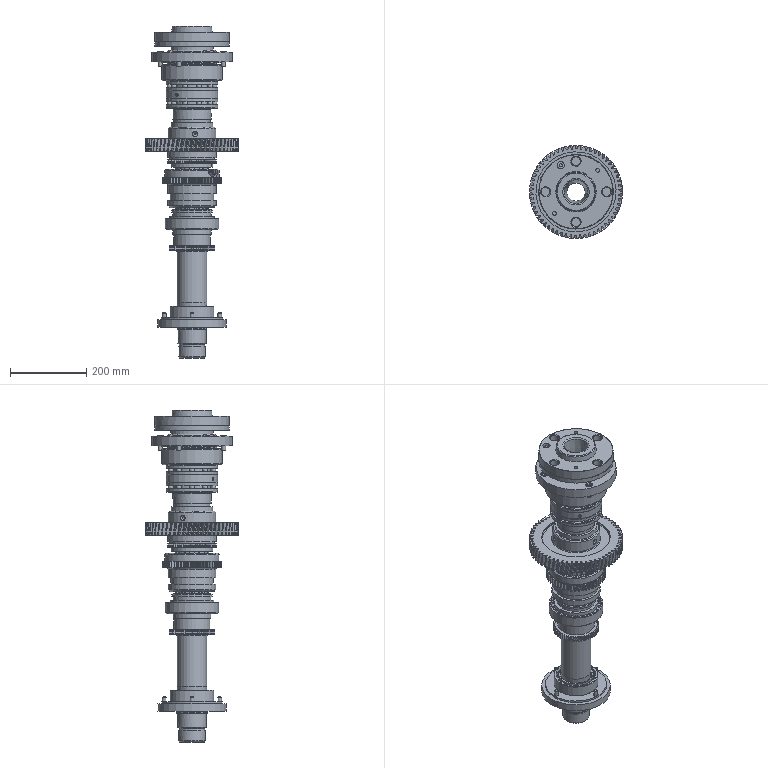Assembly | NX | mm | 30 component files | 159 solids | 2785 faces | box 243.58 x 243.58 x 869.95 mm | volume 8707448 mm3 | other 1076 | cylinder 649 | plane 589 | spline 290 | cone 101 | torus 60 | sphere 20 | commonest cylinder face diameters 119 x62 120 x58 225.579 x58 111 x58 129 x57 142.5 x50 6.667 x40 9.167 x40
Bill of materials:
unnamed part 1 | 1 |  | Annular rolling-element bearing-like assembly: outer ring, stepped inner ring, and a single circumferential row of rollers between them.
unnamed part 2 | 1 |  | Long stepped shaft with an integral circular flange at one end. The flange has a raised central boss and a through bore.
unnamed part 3 | 8 |  | Cap-screw-like part: a cylindrical head on a plain cylindrical shank with a chamfered tip.
unnamed part 4 | 1 |  | Thin-walled cylindrical sleeve with sawtooth external ridges between plain cylindrical bands at both ends.
unnamed part 5 | 1 |  | Flat annular plate with a large central hole and three small through holes in the ring area.
unnamed part 6 | 1 |  | Plain flat ring of rectangular cross-section with one small radial hole in the outer cylindrical surface.
unnamed part 7 | 1 |  | Toothed hub or sleeve: an external tooth band, fine teeth around one end face, an internally notched bore, and a stepped cylindrical body.
unnamed part 8 | 2 |  | Thrust-bearing-like assembly: two flat parallel washers separated by a single circular row of balls.
unnamed part 9 | 1 |  | Thick flat ring of rectangular cross-section with small radial holes in the outer cylindrical surface.
unnamed part 10 | 1 |  | Circular flange plate with a central bore, four equally spaced through holes, and a shallow raised face or spigot on one side.
unnamed part 11 | 1 |  | Flanged ring with an L-shaped stepped profile: a larger chamfered lip on one end and a smaller-diameter cylindrical body.
unnamed part 12 | 1 |  | Very thin flat annular washer or shim with plain inner and outer edges.
unnamed part 13 | 1 |  | Annular spur-toothed ring with a tall cylindrical collar rising from one face; large through bore with a small rectangular key-like tab projecting into the bore.
unnamed part 14 | 1 |  | Ring assembly-like body shaped like a radial ball bearing: concentric outer and inner rings with a ring of spherical elements between them.
unnamed part 15 | 1 |  | Helical gear with a hub on both sides and a central through bore; upper hub carries small radial holes, lower hub has a groove and a finely ridged band at its end.
unnamed part 16 | 1 |  | Thin flat annular ring with rectangular cross-section and a small radial hole through its outer cylindrical edge.
unnamed part 17 | 2 |  | Plain flat washer-like annular disc with a central round hole.
unnamed part 18 | 1 |  | Thin-walled cylindrical ring with several rectangular notches cut into one end face and a chamfer on that end's outer edge.
unnamed part 19 | 1 |  | Ring body shaped like a radial ball bearing: concentric outer and inner rings with evenly spaced spherical elements between them.
unnamed part 20 | 1 |  | Flat annular flange plate with four holes on a bolt circle, a stepped central bore, and a shallow pilot spigot on one face.
unnamed part 21 | 1 |  | Plain cylindrical ring/spacer with rectangular cross-section and a central through bore.
Mates:
1. touch align | CA6140-zhuzhou 1 face | CA6140-zhuzhou-yougai 1 face
2. touch align | CA6140-zhuzhou 1 face | CA6140-zhuzhou-yougai 1 face
3. touch align | CA6140-zhuzhou 1 face | CA6140-zhuzhou-yougai 1 face
4. touch align | CA6140-zhuzhou-yougai 1 face | CA6140-zhuzhou-DIANQUAN 2 face
5. touch align | CA6140-zhuzhou-yougai 1 face | CA6140-zhuzhou-DIANQUAN 1 face
6. touch align | CA6140-zhuzhou 1 face | CA6140-zhuzhou-mifeng1 1 face
7. distance | CA6140-zhuzhou-mifeng1 1 face | CA6140-zhuzhou 1 face
8. touch align | CA6140-zhuzhou 1 face | CA6140-zhuzhou-DANGYOU 1 face
9. touch align | CA6140-zhuzhou-DANGYOU 1 face | CA6140-zhuzhou 1 edge
10. touch align | CA6140-zhuzhou 1 face | CA6140-zhuzhou-DUANGAIYOU 1 face
11. touch align | CA6140-zhuzhou-DUANGAIYOU 1 face | CA6140-zhuzhou-mifeng1 1 face
12. touch align | CA6140-zhuzhou-DUANGAIYOU 1 face | CA6140-zhuzhou-luoding 8 face
13. touch align | CA6140-zhuzhou-DUANGAIYOU 1 face | CA6140-zhuzhou-luoding 8 face
14. touch align | CA6140-zhuzhou-DUANGAIYOU 1 face | CA6140-zhuzhou-luoding 7 face
15. touch align | CA6140-zhuzhou-DUANGAIYOU 1 face | CA6140-zhuzhou-luoding 7 face
16. touch align | CA6140-zhuzhou-DUANGAIYOU 1 face | CA6140-zhuzhou-luoding 6 face
17. touch align | CA6140-zhuzhou-DUANGAIYOU 1 face | CA6140-zhuzhou-luoding 6 face
18. touch align | CA6140-zhuzhou-DUANGAIYOU 1 face | CA6140-zhuzhou-luoding 5 face
19. touch align | CA6140-zhuzhou-DUANGAIYOU 1 face | CA6140-zhuzhou-luoding 5 face
20. touch align | CA6140-zhuzhou 1 face | CA6140-zhuzhou-D3182121 1 face
21. touch align | CA6140-zhuzhou-DANGYOU 1 face | CA6140-zhuzhou-D3182121 1 face
22. touch align | CA6140-zhuzhou 1 face | CA6140-zhuzhou-D8120 2 face
23. touch align | CA6140-zhuzhou 1 face | CA6140-zhuzhou-D8120 2 face
24. touch align | CA6140-zhuzhou 1 face | CA6140-zhuzhou-JINYOUHUAN 1 face
25. touch align | CA6140-zhuzhou-D8120 2 face | CA6140-zhuzhou-JINYOUHUAN 1 face
26. touch align | CA6140-zhuzhou-JINYOUHUAN 1 face | CA6140-zhuzhou-D8120 1 face
27. touch align | CA6140-zhuzhou 1 face | CA6140-zhuzhou-D8120 1 face
28. touch align | CA6140-zhuzhou 1 face | CA6140-zhuzhou-zhoutao4 1 face
29. touch align | CA6140-zhuzhou 1 edge | CA6140-zhuzhou-zhoutao4 1 face
30. touch align | CA6140-zhuzhou-zhoutao4 1 face | CA6140-zhuzhou 1 face
31. touch align | CA6140-zhuzhou 1 face | CA6140-zhuzhou-chilun3 1 face
32. touch align | CA6140-zhuzhou-zhoutao4 1 face | CA6140-zhuzhou-chilun3 1 face
33. touch align | CA6140-zhuzhou-chilun3 1 face | CA6140-zhuzhou-zhoutao3 1 face
34. touch align | CA6140-zhuzhou 1 face | CA6140-zhuzhou-zhoutao3 1 face
35. touch align | CA6140-zhuzhou 1 face | CA6140-zhuzhou-chilun2 1 face
36. distance | CA6140-zhuzhou-chilun2 1 face | CA6140-zhuzhou 1 face
37. touch align | CA6140-zhuzhou 1 face | CA6140-zhuzhou-chilun2 1 face
38. touch align | CA6140-zhuzhou-zhoutao2 1 face | CA6140-zhuzhou 1 face
39. touch align | CA6140-zhuzhou 1 face | CA6140-zhuzhou-zhoutao2 1 face
40. touch align | CA6140-zhuzhou 1 face | CA6140-zhuzhou-7516E-32216 1 face
41. touch align | CA6140-zhuzhou-7516E-32216 1 face | CA6140-zhuzhou-zhoutao2 1 face
42. touch align | CA6140-zhuzhou 1 face | CA6140-zhuzhou-zhoutao1 1 face
43. touch align | CA6140-zhuzhou-7516E-32216 1 face | CA6140-zhuzhou-zhoutao1 1 face
44. touch align | CA6140-zhuzhou 1 face | CA6140-zhuzhou-chilun1 1 face
45. touch align | CA6140-zhuzhou-zhoutao1 1 face | CA6140-zhuzhou-chilun1 1 face
46. touch align | CA6140-zhuzhou 1 face | CA6140-zhuzhou-mifengquan 1 face
47. touch align | CA6140-zhuzhou 1 face | CA6140-zhuzhou-mifengquan 1 face
48. touch align | CA6140-zhuzhou-mifengquan 1 face | CA6140-zhuzhou-E3182115 1 face
49. touch align | CA6140-zhuzhou 1 face | CA6140-zhuzhou-DUANGAIZUO 1 face
50. touch align | CA6140-zhuzhou-DUANGAIZUO 1 face | CA6140-zhuzhou-E3182115 1 face
51. touch align | CA6140-zhuzhou-DUANGAIZUO 1 face | CA6140-zhuzhou-luoding 4 face
52. touch align | CA6140-zhuzhou-DUANGAIZUO 1 face | CA6140-zhuzhou-luoding 4 face
53. touch align | CA6140-zhuzhou-DUANGAIZUO 1 face | CA6140-zhuzhou-luoding 3 face
54. touch align | CA6140-zhuzhou-DUANGAIZUO 1 face | CA6140-zhuzhou-luoding 3 face
55. touch align | CA6140-zhuzhou-DUANGAIZUO 1 face | CA6140-zhuzhou-luoding 2 face
56. touch align | CA6140-zhuzhou-DUANGAIZUO 1 face | CA6140-zhuzhou-luoding 2 face
57. touch align | CA6140-zhuzhou-DUANGAIZUO 1 face | CA6140-zhuzhou-luoding 1 face
58. touch align | CA6140-zhuzhou-DUANGAIZUO 1 face | CA6140-zhuzhou-luoding 1 face